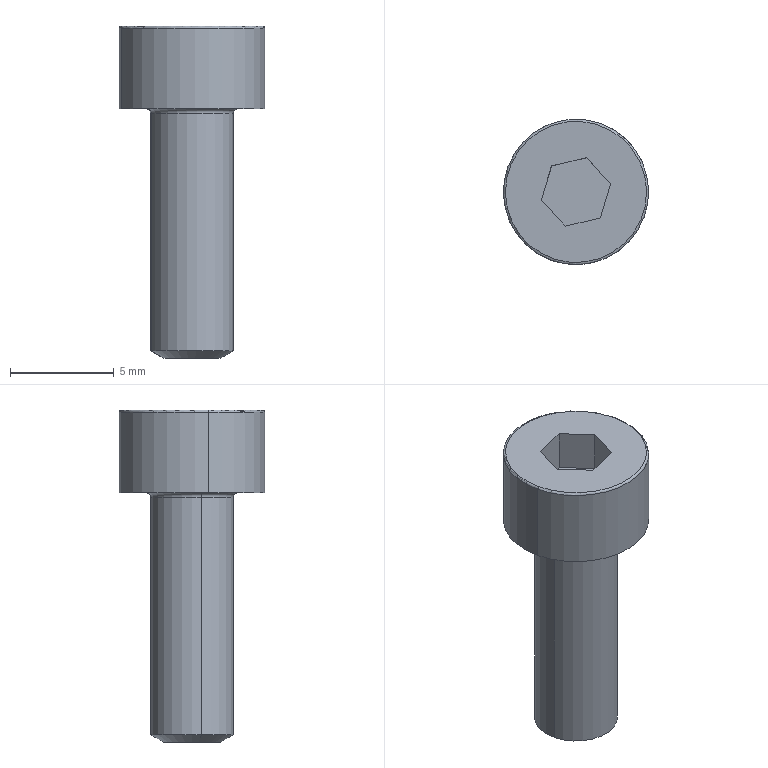Component | SolidWorks | MGL-PACK-01-00WeldedPlate1Assembly-1_SocketHeadCapScrew_M4_12[GB_T70.1-2000]-1 | 1 solid | 20 faces | box 7 x 7 x 16 mm | volume 288 mm3 | plane 10 | torus 4 | cylinder 4 | cone 2 | commonest cylinder face diameters 7 x2 4 x2
STEP:
#1=COLOUR_RGB('',0.7922,0.8196,0.9333);
#2=FILL_AREA_STYLE_COLOUR('',#1);
#3=FILL_AREA_STYLE('',(#2));
#4=SURFACE_STYLE_FILL_AREA(#3);
#5=SURFACE_SIDE_STYLE('',(#4));
#6=SURFACE_STYLE_USAGE(.BOTH.,#5);
#7=PRESENTATION_STYLE_ASSIGNMENT((#6));
#8=CARTESIAN_POINT('',(3.416,-2.272,0.3543));
#9=VERTEX_POINT('',#8);
#10=CARTESIAN_POINT('',(3.155,-2.334,0.3543));
#11=VERTEX_POINT('',#10);
#12=CARTESIAN_POINT('',(3.285,-2.303,0.3543));
#13=DIRECTION('',(0.,-0.,1.));
#14=DIRECTION('',(-0.9734,-0.2292,0.));
#15=AXIS2_PLACEMENT_3D('',#12,#13,#14);
#16=CIRCLE('',#15,0.1339);
#17=EDGE_CURVE('',#9,#11,#16,.T.);
#18=ORIENTED_EDGE('',*,*,#17,.F.);
#19=CARTESIAN_POINT('',(3.42,-2.272,0.3504));
#20=VERTEX_POINT('',#19);
#21=CARTESIAN_POINT('',(3.416,-2.272,0.3504));
#22=DIRECTION('',(-0.2292,0.9734,0.));
#23=DIRECTION('',(-0.9734,-0.2292,0.));
#24=AXIS2_PLACEMENT_3D('',#21,#22,#23);
#25=CIRCLE('',#24,0.003937);
#26=EDGE_CURVE('',#9,#20,#25,.T.);
#27=ORIENTED_EDGE('',*,*,#26,.T.);
#28=CARTESIAN_POINT('',(3.151,-2.335,0.3504));
#29=VERTEX_POINT('',#28);
#30=CARTESIAN_POINT('',(3.285,-2.303,0.3504));
#31=DIRECTION('',(0.,0.,-1.));
#32=DIRECTION('',(-0.9734,-0.2292,0.));
#33=AXIS2_PLACEMENT_3D('',#30,#31,#32);
#34=CIRCLE('',#33,0.1378);
#35=EDGE_CURVE('',#29,#20,#34,.T.);
#36=ORIENTED_EDGE('',*,*,#35,.F.);
#37=CARTESIAN_POINT('',(3.155,-2.334,0.3504));
#38=DIRECTION('',(0.2292,-0.9734,-0.));
#39=DIRECTION('',(0.9734,0.2292,0.));
#40=AXIS2_PLACEMENT_3D('',#37,#38,#39);
#41=CIRCLE('',#40,0.003937);
#42=EDGE_CURVE('',#11,#29,#41,.T.);
#43=ORIENTED_EDGE('',*,*,#42,.F.);
#44=EDGE_LOOP('',(#18,#27,#36,#43));
#45=FACE_OUTER_BOUND('',#44,.T.);
#46=CARTESIAN_POINT('',(3.285,-2.303,0.3504));
#47=DIRECTION('',(0.,0.,-1.));
#48=DIRECTION('',(-0.9734,-0.2292,-0.));
#49=AXIS2_PLACEMENT_3D('',#46,#47,#48);
#50=TOROIDAL_SURFACE('',#49,0.1339,0.003937);
#51=ADVANCED_FACE('',(#45),#50,.T.);
#52=CARTESIAN_POINT('',(3.339,-2.291,-0.2756));
#53=VERTEX_POINT('',#52);
#54=CARTESIAN_POINT('',(3.232,-2.316,-0.2756));
#55=VERTEX_POINT('',#54);
#56=CARTESIAN_POINT('',(3.285,-2.303,-0.2756));
#57=DIRECTION('',(0.,-0.,1.));
#58=DIRECTION('',(0.9734,0.2292,0.));
#59=AXIS2_PLACEMENT_3D('',#56,#57,#58);
#60=CIRCLE('',#59,0.05487);
#61=EDGE_CURVE('',#53,#55,#60,.T.);
#62=ORIENTED_EDGE('',*,*,#61,.T.);
#63=CARTESIAN_POINT('',(3.209,-2.321,-0.2618));
#64=VERTEX_POINT('',#63);
#65=CARTESIAN_POINT('',(3.209,-2.321,-0.2618));
#66=DIRECTION('',(-0.843,-0.1985,0.5));
#67=VECTOR('',#66,39.37);
#68=LINE('',#65,#67);
#69=EDGE_CURVE('',#55,#64,#68,.T.);
#70=ORIENTED_EDGE('',*,*,#69,.T.);
#71=CARTESIAN_POINT('',(3.362,-2.285,-0.2618));
#72=VERTEX_POINT('',#71);
#73=CARTESIAN_POINT('',(3.285,-2.303,-0.2618));
#74=DIRECTION('',(0.,-0.,1.));
#75=DIRECTION('',(0.9734,0.2292,0.));
#76=AXIS2_PLACEMENT_3D('',#73,#74,#75);
#77=CIRCLE('',#76,0.07874);
#78=EDGE_CURVE('',#72,#64,#77,.T.);
#79=ORIENTED_EDGE('',*,*,#78,.F.);
#80=CARTESIAN_POINT('',(3.362,-2.285,-0.2618));
#81=DIRECTION('',(0.843,0.1985,0.5));
#82=VECTOR('',#81,39.37);
#83=LINE('',#80,#82);
#84=EDGE_CURVE('',#53,#72,#83,.T.);
#85=ORIENTED_EDGE('',*,*,#84,.F.);
#86=EDGE_LOOP('',(#62,#70,#79,#85));
#87=FACE_OUTER_BOUND('',#86,.T.);
#88=CARTESIAN_POINT('',(3.285,-2.303,-0.2618));
#89=DIRECTION('',(0.,-0.,1.));
#90=DIRECTION('',(0.9734,0.2292,0.));
#91=AXIS2_PLACEMENT_3D('',#88,#89,#90);
#92=CONICAL_SURFACE('',#91,0.07874,1.047);
#93=ADVANCED_FACE('',(#87),#92,.T.);
#94=CARTESIAN_POINT('',(3.201,-2.323,0.1969));
#95=VERTEX_POINT('',#94);
#96=CARTESIAN_POINT('',(3.37,-2.283,0.1969));
#97=VERTEX_POINT('',#96);
#98=CARTESIAN_POINT('',(3.285,-2.303,0.1969));
#99=DIRECTION('',(0.,-0.,1.));
#100=DIRECTION('',(0.9734,0.2292,0.));
#101=AXIS2_PLACEMENT_3D('',#98,#99,#100);
#102=CIRCLE('',#101,0.08661);
#103=EDGE_CURVE('',#95,#97,#102,.T.);
#104=ORIENTED_EDGE('',*,*,#103,.F.);
#105=CARTESIAN_POINT('',(3.209,-2.321,0.189));
#106=VERTEX_POINT('',#105);
#107=CARTESIAN_POINT('',(3.201,-2.323,0.189));
#108=DIRECTION('',(-0.2292,0.9734,0.));
#109=DIRECTION('',(-0.9734,-0.2292,0.));
#110=AXIS2_PLACEMENT_3D('',#107,#108,#109);
#111=CIRCLE('',#110,0.007874);
#112=EDGE_CURVE('',#95,#106,#111,.T.);
#113=ORIENTED_EDGE('',*,*,#112,.T.);
#114=CARTESIAN_POINT('',(3.362,-2.285,0.189));
#115=VERTEX_POINT('',#114);
#116=CARTESIAN_POINT('',(3.285,-2.303,0.189));
#117=DIRECTION('',(0.,-0.,1.));
#118=DIRECTION('',(0.9734,0.2292,0.));
#119=AXIS2_PLACEMENT_3D('',#116,#117,#118);
#120=CIRCLE('',#119,0.07874);
#121=EDGE_CURVE('',#106,#115,#120,.T.);
#122=ORIENTED_EDGE('',*,*,#121,.T.);
#123=CARTESIAN_POINT('',(3.37,-2.283,0.189));
#124=DIRECTION('',(0.2292,-0.9734,-0.));
#125=DIRECTION('',(0.9734,0.2292,0.));
#126=AXIS2_PLACEMENT_3D('',#123,#124,#125);
#127=CIRCLE('',#126,0.007874);
#128=EDGE_CURVE('',#97,#115,#127,.T.);
#129=ORIENTED_EDGE('',*,*,#128,.F.);
#130=EDGE_LOOP('',(#104,#113,#122,#129));
#131=FACE_OUTER_BOUND('',#130,.T.);
#132=CARTESIAN_POINT('',(3.285,-2.303,0.189));
#133=DIRECTION('',(0.,-0.,1.));
#134=DIRECTION('',(0.9734,0.2292,0.));
#135=AXIS2_PLACEMENT_3D('',#132,#133,#134);
#136=TOROIDAL_SURFACE('',#135,0.08661,0.007874);
#137=ADVANCED_FACE('',(#131),#136,.F.);
#138=CARTESIAN_POINT('',(3.42,-2.272,0.1969));
#139=VERTEX_POINT('',#138);
#140=CARTESIAN_POINT('',(3.151,-2.335,0.1969));
#141=VERTEX_POINT('',#140);
#142=CARTESIAN_POINT('',(3.285,-2.303,0.1969));
#143=DIRECTION('',(0.,-0.,1.));
#144=DIRECTION('',(0.9734,0.2292,0.));
#145=AXIS2_PLACEMENT_3D('',#142,#143,#144);
#146=CIRCLE('',#145,0.1378);
#147=EDGE_CURVE('',#139,#141,#146,.T.);
#148=ORIENTED_EDGE('',*,*,#147,.T.);
#149=CARTESIAN_POINT('',(3.151,-2.335,0.3543));
#150=DIRECTION('',(0.,-0.,1.));
#151=VECTOR('',#150,39.37);
#152=LINE('',#149,#151);
#153=EDGE_CURVE('',#141,#29,#152,.T.);
#154=ORIENTED_EDGE('',*,*,#153,.T.);
#155=ORIENTED_EDGE('',*,*,#35,.T.);
#156=CARTESIAN_POINT('',(3.42,-2.272,0.3543));
#157=DIRECTION('',(0.,-0.,1.));
#158=VECTOR('',#157,39.37);
#159=LINE('',#156,#158);
#160=EDGE_CURVE('',#139,#20,#159,.T.);
#161=ORIENTED_EDGE('',*,*,#160,.F.);
#162=EDGE_LOOP('',(#148,#154,#155,#161));
#163=FACE_OUTER_BOUND('',#162,.T.);
#164=CARTESIAN_POINT('',(3.285,-2.303,0.3543));
#165=DIRECTION('',(0.,-0.,1.));
#166=DIRECTION('',(0.9734,0.2292,0.));
#167=AXIS2_PLACEMENT_3D('',#164,#165,#166);
#168=CYLINDRICAL_SURFACE('',#167,0.1378);
#169=ADVANCED_FACE('',(#163),#168,.T.);
#170=ORIENTED_EDGE('',*,*,#78,.T.);
#171=CARTESIAN_POINT('',(3.209,-2.321,0.3543));
#172=DIRECTION('',(0.,-0.,1.));
#173=VECTOR('',#172,39.37);
#174=LINE('',#171,#173);
#175=EDGE_CURVE('',#64,#106,#174,.T.);
#176=ORIENTED_EDGE('',*,*,#175,.T.);
#177=CARTESIAN_POINT('',(3.285,-2.303,0.189));
#178=DIRECTION('',(0.,-0.,1.));
#179=DIRECTION('',(0.9734,0.2292,0.));
#180=AXIS2_PLACEMENT_3D('',#177,#178,#179);
#181=CIRCLE('',#180,0.07874);
#182=EDGE_CURVE('',#115,#106,#181,.T.);
#183=ORIENTED_EDGE('',*,*,#182,.F.);
#184=CARTESIAN_POINT('',(3.362,-2.285,0.3543));
#185=DIRECTION('',(0.,-0.,1.));
#186=VECTOR('',#185,39.37);
#187=LINE('',#184,#186);
#188=EDGE_CURVE('',#72,#115,#187,.T.);
#189=ORIENTED_EDGE('',*,*,#188,.F.);
#190=EDGE_LOOP('',(#170,#176,#183,#189));
#191=FACE_OUTER_BOUND('',#190,.T.);
#192=CARTESIAN_POINT('',(3.285,-2.303,0.3543));
#193=DIRECTION('',(0.,-0.,1.));
#194=DIRECTION('',(0.9734,0.2292,0.));
#195=AXIS2_PLACEMENT_3D('',#192,#193,#194);
#196=CYLINDRICAL_SURFACE('',#195,0.07874);
#197=ADVANCED_FACE('',(#191),#196,.T.);
#198=ORIENTED_EDGE('',*,*,#175,.F.);
#199=CARTESIAN_POINT('',(3.285,-2.303,-0.2618));
#200=DIRECTION('',(0.,-0.,1.));
#201=DIRECTION('',(0.9734,0.2292,0.));
#202=AXIS2_PLACEMENT_3D('',#199,#200,#201);
#203=CIRCLE('',#202,0.07874);
#204=EDGE_CURVE('',#64,#72,#203,.T.);
#205=ORIENTED_EDGE('',*,*,#204,.T.);
#206=ORIENTED_EDGE('',*,*,#188,.T.);
#207=ORIENTED_EDGE('',*,*,#121,.F.);
#208=EDGE_LOOP('',(#198,#205,#206,#207));
#209=FACE_OUTER_BOUND('',#208,.T.);
#210=CARTESIAN_POINT('',(3.285,-2.303,0.3543));
#211=DIRECTION('',(0.,-0.,1.));
#212=DIRECTION('',(0.9734,0.2292,0.));
#213=AXIS2_PLACEMENT_3D('',#210,#211,#212);
#214=CYLINDRICAL_SURFACE('',#213,0.07874);
#215=ADVANCED_FACE('',(#209),#214,.T.);
#216=CARTESIAN_POINT('',(3.285,-2.303,0.3543));
#217=DIRECTION('',(0.,-0.,1.));
#218=DIRECTION('',(-0.9734,-0.2292,0.));
#219=AXIS2_PLACEMENT_3D('',#216,#217,#218);
#220=CIRCLE('',#219,0.1339);
#221=EDGE_CURVE('',#11,#9,#220,.T.);
#222=ORIENTED_EDGE('',*,*,#221,.T.);
#223=ORIENTED_EDGE('',*,*,#17,.T.);
#224=EDGE_LOOP('',(#222,#223));
#225=FACE_OUTER_BOUND('',#224,.T.);
#226=CARTESIAN_POINT('',(3.351,-2.288,0.3543));
#227=VERTEX_POINT('',#226);
#228=CARTESIAN_POINT('',(3.305,-2.238,0.3543));
#229=VERTEX_POINT('',#228);
#230=CARTESIAN_POINT('',(3.351,-2.288,0.3543));
#231=DIRECTION('',(-0.6852,0.7284,-0.));
#232=VECTOR('',#231,39.37);
#233=LINE('',#230,#232);
#234=EDGE_CURVE('',#227,#229,#233,.T.);
#235=ORIENTED_EDGE('',*,*,#234,.F.);
#236=CARTESIAN_POINT('',(3.332,-2.352,0.3543));
#237=VERTEX_POINT('',#236);
#238=CARTESIAN_POINT('',(3.332,-2.352,0.3543));
#239=DIRECTION('',(0.2882,0.9576,0.));
#240=VECTOR('',#239,39.37);
#241=LINE('',#238,#240);
#242=EDGE_CURVE('',#237,#227,#241,.T.);
#243=ORIENTED_EDGE('',*,*,#242,.F.);
#244=CARTESIAN_POINT('',(3.266,-2.368,0.3543));
#245=VERTEX_POINT('',#244);
#246=CARTESIAN_POINT('',(3.266,-2.368,0.3543));
#247=DIRECTION('',(0.9734,0.2292,0.));
#248=VECTOR('',#247,39.37);
#249=LINE('',#246,#248);
#250=EDGE_CURVE('',#245,#237,#249,.T.);
#251=ORIENTED_EDGE('',*,*,#250,.F.);
#252=CARTESIAN_POINT('',(3.22,-2.319,0.3543));
#253=VERTEX_POINT('',#252);
#254=CARTESIAN_POINT('',(3.22,-2.319,0.3543));
#255=DIRECTION('',(0.6852,-0.7284,0.));
#256=VECTOR('',#255,39.37);
#257=LINE('',#254,#256);
#258=EDGE_CURVE('',#253,#245,#257,.T.);
#259=ORIENTED_EDGE('',*,*,#258,.F.);
#260=CARTESIAN_POINT('',(3.239,-2.254,0.3543));
#261=VERTEX_POINT('',#260);
#262=CARTESIAN_POINT('',(3.239,-2.254,0.3543));
#263=DIRECTION('',(-0.2882,-0.9576,-0.));
#264=VECTOR('',#263,39.37);
#265=LINE('',#262,#264);
#266=EDGE_CURVE('',#261,#253,#265,.T.);
#267=ORIENTED_EDGE('',*,*,#266,.F.);
#268=CARTESIAN_POINT('',(3.305,-2.238,0.3543));
#269=DIRECTION('',(-0.9734,-0.2292,-0.));
#270=VECTOR('',#269,39.37);
#271=LINE('',#268,#270);
#272=EDGE_CURVE('',#229,#261,#271,.T.);
#273=ORIENTED_EDGE('',*,*,#272,.F.);
#274=EDGE_LOOP('',(#235,#243,#251,#259,#267,#273));
#275=FACE_BOUND('',#274,.T.);
#276=CARTESIAN_POINT('',(3.285,-2.303,0.3543));
#277=DIRECTION('',(0.,0.,-1.));
#278=DIRECTION('',(-0.9734,-0.2292,-0.));
#279=AXIS2_PLACEMENT_3D('',#276,#277,#278);
#280=PLANE('',#279);
#281=ADVANCED_FACE('',(#225,#275),#280,.F.);
#282=ORIENTED_EDGE('',*,*,#153,.F.);
#283=CARTESIAN_POINT('',(3.285,-2.303,0.1969));
#284=DIRECTION('',(0.,-0.,1.));
#285=DIRECTION('',(0.9734,0.2292,0.));
#286=AXIS2_PLACEMENT_3D('',#283,#284,#285);
#287=CIRCLE('',#286,0.1378);
#288=EDGE_CURVE('',#141,#139,#287,.T.);
#289=ORIENTED_EDGE('',*,*,#288,.T.);
#290=ORIENTED_EDGE('',*,*,#160,.T.);
#291=CARTESIAN_POINT('',(3.285,-2.303,0.3504));
#292=DIRECTION('',(0.,0.,-1.));
#293=DIRECTION('',(-0.9734,-0.2292,0.));
#294=AXIS2_PLACEMENT_3D('',#291,#292,#293);
#295=CIRCLE('',#294,0.1378);
#296=EDGE_CURVE('',#20,#29,#295,.T.);
#297=ORIENTED_EDGE('',*,*,#296,.T.);
#298=EDGE_LOOP('',(#282,#289,#290,#297));
#299=FACE_OUTER_BOUND('',#298,.T.);
#300=CARTESIAN_POINT('',(3.285,-2.303,0.3543));
#301=DIRECTION('',(0.,-0.,1.));
#302=DIRECTION('',(0.9734,0.2292,0.));
#303=AXIS2_PLACEMENT_3D('',#300,#301,#302);
#304=CYLINDRICAL_SURFACE('',#303,0.1378);
#305=ADVANCED_FACE('',(#299),#304,.T.);
#306=ORIENTED_EDGE('',*,*,#147,.F.);
#307=ORIENTED_EDGE('',*,*,#288,.F.);
#308=EDGE_LOOP('',(#306,#307));
#309=FACE_OUTER_BOUND('',#308,.T.);
#310=CARTESIAN_POINT('',(3.285,-2.303,0.1969));
#311=DIRECTION('',(0.,-0.,1.));
#312=DIRECTION('',(0.9734,0.2292,0.));
#313=AXIS2_PLACEMENT_3D('',#310,#311,#312);
#314=CIRCLE('',#313,0.08661);
#315=EDGE_CURVE('',#97,#95,#314,.T.);
#316=ORIENTED_EDGE('',*,*,#315,.T.);
#317=ORIENTED_EDGE('',*,*,#103,.T.);
#318=EDGE_LOOP('',(#316,#317));
#319=FACE_BOUND('',#318,.T.);
#320=CARTESIAN_POINT('',(3.254,-2.169,0.1969));
#321=DIRECTION('',(-0.,-0.,1.));
#322=DIRECTION('',(0.9734,0.2292,0.));
#323=AXIS2_PLACEMENT_3D('',#320,#321,#322);
#324=PLANE('',#323);
#325=ADVANCED_FACE('',(#309,#319),#324,.F.);
#326=ORIENTED_EDGE('',*,*,#112,.F.);
#327=ORIENTED_EDGE('',*,*,#315,.F.);
#328=ORIENTED_EDGE('',*,*,#128,.T.);
#329=ORIENTED_EDGE('',*,*,#182,.T.);
#330=EDGE_LOOP('',(#326,#327,#328,#329));
#331=FACE_OUTER_BOUND('',#330,.T.);
#332=CARTESIAN_POINT('',(3.285,-2.303,0.189));
#333=DIRECTION('',(0.,-0.,1.));
#334=DIRECTION('',(0.9734,0.2292,0.));
#335=AXIS2_PLACEMENT_3D('',#332,#333,#334);
#336=TOROIDAL_SURFACE('',#335,0.08661,0.007874);
#337=ADVANCED_FACE('',(#331),#336,.F.);
#338=ORIENTED_EDGE('',*,*,#242,.T.);
#339=CARTESIAN_POINT('',(3.351,-2.288,0.2756));
#340=VERTEX_POINT('',#339);
#341=CARTESIAN_POINT('',(3.351,-2.288,0.2756));
#342=DIRECTION('',(0.,-0.,1.));
#343=VECTOR('',#342,39.37);
#344=LINE('',#341,#343);
#345=EDGE_CURVE('',#340,#227,#344,.T.);
#346=ORIENTED_EDGE('',*,*,#345,.F.);
#347=CARTESIAN_POINT('',(3.332,-2.352,0.2756));
#348=VERTEX_POINT('',#347);
#349=CARTESIAN_POINT('',(3.332,-2.352,0.2756));
#350=DIRECTION('',(0.2882,0.9576,0.));
#351=VECTOR('',#350,39.37);
#352=LINE('',#349,#351);
#353=EDGE_CURVE('',#348,#340,#352,.T.);
#354=ORIENTED_EDGE('',*,*,#353,.F.);
#355=CARTESIAN_POINT('',(3.332,-2.352,0.2756));
#356=DIRECTION('',(0.,-0.,1.));
#357=VECTOR('',#356,39.37);
#358=LINE('',#355,#357);
#359=EDGE_CURVE('',#348,#237,#358,.T.);
#360=ORIENTED_EDGE('',*,*,#359,.T.);
#361=EDGE_LOOP('',(#338,#346,#354,#360));
#362=FACE_OUTER_BOUND('',#361,.T.);
#363=CARTESIAN_POINT('',(3.332,-2.352,0.2756));
#364=DIRECTION('',(0.9576,-0.2882,0.));
#365=DIRECTION('',(-0.2882,-0.9576,-0.));
#366=AXIS2_PLACEMENT_3D('',#363,#364,#365);
#367=PLANE('',#366);
#368=ADVANCED_FACE('',(#362),#367,.F.);
#369=ORIENTED_EDGE('',*,*,#250,.T.);
#370=ORIENTED_EDGE('',*,*,#359,.F.);
#371=CARTESIAN_POINT('',(3.266,-2.368,0.2756));
#372=VERTEX_POINT('',#371);
#373=CARTESIAN_POINT('',(3.266,-2.368,0.2756));
#374=DIRECTION('',(0.9734,0.2292,0.));
#375=VECTOR('',#374,39.37);
#376=LINE('',#373,#375);
#377=EDGE_CURVE('',#372,#348,#376,.T.);
#378=ORIENTED_EDGE('',*,*,#377,.F.);
#379=CARTESIAN_POINT('',(3.266,-2.368,0.2756));
#380=DIRECTION('',(0.,-0.,1.));
#381=VECTOR('',#380,39.37);
#382=LINE('',#379,#381);
#383=EDGE_CURVE('',#372,#245,#382,.T.);
#384=ORIENTED_EDGE('',*,*,#383,.T.);
#385=EDGE_LOOP('',(#369,#370,#378,#384));
#386=FACE_OUTER_BOUND('',#385,.T.);
#387=CARTESIAN_POINT('',(3.266,-2.368,0.2756));
#388=DIRECTION('',(0.2292,-0.9734,0.));
#389=DIRECTION('',(-0.9734,-0.2292,-0.));
#390=AXIS2_PLACEMENT_3D('',#387,#388,#389);
#391=PLANE('',#390);
#392=ADVANCED_FACE('',(#386),#391,.F.);
#393=ORIENTED_EDGE('',*,*,#258,.T.);
#394=ORIENTED_EDGE('',*,*,#383,.F.);
#395=CARTESIAN_POINT('',(3.22,-2.319,0.2756));
#396=VERTEX_POINT('',#395);
#397=CARTESIAN_POINT('',(3.22,-2.319,0.2756));
#398=DIRECTION('',(0.6852,-0.7284,0.));
#399=VECTOR('',#398,39.37);
#400=LINE('',#397,#399);
#401=EDGE_CURVE('',#396,#372,#400,.T.);
#402=ORIENTED_EDGE('',*,*,#401,.F.);
#403=CARTESIAN_POINT('',(3.22,-2.319,0.2756));
#404=DIRECTION('',(0.,-0.,1.));
#405=VECTOR('',#404,39.37);
#406=LINE('',#403,#405);
#407=EDGE_CURVE('',#396,#253,#406,.T.);
#408=ORIENTED_EDGE('',*,*,#407,.T.);
#409=EDGE_LOOP('',(#393,#394,#402,#408));
#410=FACE_OUTER_BOUND('',#409,.T.);
#411=CARTESIAN_POINT('',(3.22,-2.319,0.2756));
#412=DIRECTION('',(-0.7284,-0.6852,-0.));
#413=DIRECTION('',(-0.6852,0.7284,-0.));
#414=AXIS2_PLACEMENT_3D('',#411,#412,#413);
#415=PLANE('',#414);
#416=ADVANCED_FACE('',(#410),#415,.F.);
#417=ORIENTED_EDGE('',*,*,#266,.T.);
#418=ORIENTED_EDGE('',*,*,#407,.F.);
#419=CARTESIAN_POINT('',(3.239,-2.254,0.2756));
#420=VERTEX_POINT('',#419);
#421=CARTESIAN_POINT('',(3.239,-2.254,0.2756));
#422=DIRECTION('',(-0.2882,-0.9576,-0.));
#423=VECTOR('',#422,39.37);
#424=LINE('',#421,#423);
#425=EDGE_CURVE('',#420,#396,#424,.T.);
#426=ORIENTED_EDGE('',*,*,#425,.F.);
#427=CARTESIAN_POINT('',(3.239,-2.254,0.2756));
#428=DIRECTION('',(0.,-0.,1.));
#429=VECTOR('',#428,39.37);
#430=LINE('',#427,#429);
#431=EDGE_CURVE('',#420,#261,#430,.T.);
#432=ORIENTED_EDGE('',*,*,#431,.T.);
#433=EDGE_LOOP('',(#417,#418,#426,#432));
#434=FACE_OUTER_BOUND('',#433,.T.);
#435=CARTESIAN_POINT('',(3.239,-2.254,0.2756));
#436=DIRECTION('',(-0.9576,0.2882,-0.));
#437=DIRECTION('',(0.2882,0.9576,0.));
#438=AXIS2_PLACEMENT_3D('',#435,#436,#437);
#439=PLANE('',#438);
#440=ADVANCED_FACE('',(#434),#439,.F.);
#441=ORIENTED_EDGE('',*,*,#272,.T.);
#442=ORIENTED_EDGE('',*,*,#431,.F.);
#443=CARTESIAN_POINT('',(3.305,-2.238,0.2756));
#444=VERTEX_POINT('',#443);
#445=CARTESIAN_POINT('',(3.305,-2.238,0.2756));
#446=DIRECTION('',(-0.9734,-0.2292,-0.));
#447=VECTOR('',#446,39.37);
#448=LINE('',#445,#447);
#449=EDGE_CURVE('',#444,#420,#448,.T.);
#450=ORIENTED_EDGE('',*,*,#449,.F.);
#451=CARTESIAN_POINT('',(3.305,-2.238,0.2756));
#452=DIRECTION('',(0.,-0.,1.));
#453=VECTOR('',#452,39.37);
#454=LINE('',#451,#453);
#455=EDGE_CURVE('',#444,#229,#454,.T.);
#456=ORIENTED_EDGE('',*,*,#455,.T.);
#457=EDGE_LOOP('',(#441,#442,#450,#456));
#458=FACE_OUTER_BOUND('',#457,.T.);
#459=CARTESIAN_POINT('',(3.305,-2.238,0.2756));
#460=DIRECTION('',(-0.2292,0.9734,0.));
#461=DIRECTION('',(0.9734,0.2292,0.));
#462=AXIS2_PLACEMENT_3D('',#459,#460,#461);
#463=PLANE('',#462);
#464=ADVANCED_FACE('',(#458),#463,.F.);
#465=ORIENTED_EDGE('',*,*,#234,.T.);
#466=ORIENTED_EDGE('',*,*,#455,.F.);
#467=CARTESIAN_POINT('',(3.351,-2.288,0.2756));
#468=DIRECTION('',(-0.6852,0.7284,-0.));
#469=VECTOR('',#468,39.37);
#470=LINE('',#467,#469);
#471=EDGE_CURVE('',#340,#444,#470,.T.);
#472=ORIENTED_EDGE('',*,*,#471,.F.);
#473=ORIENTED_EDGE('',*,*,#345,.T.);
#474=EDGE_LOOP('',(#465,#466,#472,#473));
#475=FACE_OUTER_BOUND('',#474,.T.);
#476=CARTESIAN_POINT('',(3.351,-2.288,0.2756));
#477=DIRECTION('',(0.7284,0.6852,0.));
#478=DIRECTION('',(0.6852,-0.7284,0.));
#479=AXIS2_PLACEMENT_3D('',#476,#477,#478);
#480=PLANE('',#479);
#481=ADVANCED_FACE('',(#475),#480,.F.);
#482=ORIENTED_EDGE('',*,*,#353,.T.);
#483=ORIENTED_EDGE('',*,*,#471,.T.);
#484=ORIENTED_EDGE('',*,*,#449,.T.);
#485=ORIENTED_EDGE('',*,*,#425,.T.);
#486=ORIENTED_EDGE('',*,*,#401,.T.);
#487=ORIENTED_EDGE('',*,*,#377,.T.);
#488=EDGE_LOOP('',(#482,#483,#484,#485,#486,#487));
#489=FACE_OUTER_BOUND('',#488,.T.);
#490=CARTESIAN_POINT('',(3.371,-2.223,0.2756));
#491=DIRECTION('',(-0.,-0.,1.));
#492=DIRECTION('',(0.9734,0.2292,0.));
#493=AXIS2_PLACEMENT_3D('',#490,#491,#492);
#494=PLANE('',#493);
#495=ADVANCED_FACE('',(#489),#494,.T.);
#496=ORIENTED_EDGE('',*,*,#69,.F.);
#497=CARTESIAN_POINT('',(3.285,-2.303,-0.2756));
#498=DIRECTION('',(0.,-0.,1.));
#499=DIRECTION('',(0.9734,0.2292,0.));
#500=AXIS2_PLACEMENT_3D('',#497,#498,#499);
#501=CIRCLE('',#500,0.05487);
#502=EDGE_CURVE('',#55,#53,#501,.T.);
#503=ORIENTED_EDGE('',*,*,#502,.T.);
#504=ORIENTED_EDGE('',*,*,#84,.T.);
#505=ORIENTED_EDGE('',*,*,#204,.F.);
#506=EDGE_LOOP('',(#496,#503,#504,#505));
#507=FACE_OUTER_BOUND('',#506,.T.);
#508=CARTESIAN_POINT('',(3.285,-2.303,-0.2618));
#509=DIRECTION('',(0.,-0.,1.));
#510=DIRECTION('',(0.9734,0.2292,0.));
#511=AXIS2_PLACEMENT_3D('',#508,#509,#510);
#512=CONICAL_SURFACE('',#511,0.07874,1.047);
#513=ADVANCED_FACE('',(#507),#512,.T.);
#514=ORIENTED_EDGE('',*,*,#61,.F.);
#515=ORIENTED_EDGE('',*,*,#502,.F.);
#516=EDGE_LOOP('',(#514,#515));
#517=FACE_OUTER_BOUND('',#516,.T.);
#518=CARTESIAN_POINT('',(3.267,-2.227,-0.2756));
#519=DIRECTION('',(-0.,-0.,1.));
#520=DIRECTION('',(0.9734,0.2292,0.));
#521=AXIS2_PLACEMENT_3D('',#518,#519,#520);
#522=PLANE('',#521);
#523=ADVANCED_FACE('',(#517),#522,.F.);
#524=ORIENTED_EDGE('',*,*,#26,.F.);
#525=ORIENTED_EDGE('',*,*,#221,.F.);
#526=ORIENTED_EDGE('',*,*,#42,.T.);
#527=ORIENTED_EDGE('',*,*,#296,.F.);
#528=EDGE_LOOP('',(#524,#525,#526,#527));
#529=FACE_OUTER_BOUND('',#528,.T.);
#530=CARTESIAN_POINT('',(3.285,-2.303,0.3504));
#531=DIRECTION('',(0.,0.,-1.));
#532=DIRECTION('',(-0.9734,-0.2292,-0.));
#533=AXIS2_PLACEMENT_3D('',#530,#531,#532);
#534=TOROIDAL_SURFACE('',#533,0.1339,0.003937);
#535=ADVANCED_FACE('',(#529),#534,.T.);
#536=CLOSED_SHELL('',(#51,#93,#137,#169,#197,#215,#281,#305,#325,#337,#368,#392,#416,#440,#464,#481,#495,#513,#523,#535));
#537=MANIFOLD_SOLID_BREP('',#536);
#538=STYLED_ITEM('',(#7),#537);
#539=PRESENTATION_LAYER_ASSIGNMENT('','',(#538));
#540=CARTESIAN_POINT('',(0.,0.,0.));
#541=DIRECTION('',(0.,0.,1.));
#542=DIRECTION('',(1.,0.,0.));
#543=AXIS2_PLACEMENT_3D('',#540,#541,#542);
#544=(LENGTH_UNIT()NAMED_UNIT(*)SI_UNIT($,.METRE.));
#545=LENGTH_MEASURE_WITH_UNIT(LENGTH_MEASURE(0.0254),#544);
#546=DIMENSIONAL_EXPONENTS(1.,0.,0.,0.,0.,0.,0.);
#547=(CONVERSION_BASED_UNIT('',#545)LENGTH_UNIT()NAMED_UNIT(#546));
#548=UNCERTAINTY_MEASURE_WITH_UNIT(LENGTH_MEASURE(0.00001),#547,'','');
#549=(NAMED_UNIT(*)PLANE_ANGLE_UNIT()SI_UNIT($,.RADIAN.));
#550=(NAMED_UNIT(*)SI_UNIT($,.STERADIAN.)SOLID_ANGLE_UNIT());
#551=(GEOMETRIC_REPRESENTATION_CONTEXT(3)GLOBAL_UNCERTAINTY_ASSIGNED_CONTEXT((#548))GLOBAL_UNIT_ASSIGNED_CONTEXT((#547,#549,#550))REPRESENTATION_CONTEXT('',''));
#552=ADVANCED_BREP_SHAPE_REPRESENTATION('',(#537,#543),#551);
#553=(LENGTH_UNIT()NAMED_UNIT(*)SI_UNIT($,.METRE.));
#554=LENGTH_MEASURE_WITH_UNIT(LENGTH_MEASURE(0.0254),#553);
#555=DIMENSIONAL_EXPONENTS(1.,0.,0.,0.,0.,0.,0.);
#556=(CONVERSION_BASED_UNIT('',#554)LENGTH_UNIT()NAMED_UNIT(#555));
#557=UNCERTAINTY_MEASURE_WITH_UNIT(LENGTH_MEASURE(0.00001),#556,'','');
#558=(NAMED_UNIT(*)PLANE_ANGLE_UNIT()SI_UNIT($,.RADIAN.));
#559=(NAMED_UNIT(*)SI_UNIT($,.STERADIAN.)SOLID_ANGLE_UNIT());
#560=(GEOMETRIC_REPRESENTATION_CONTEXT(3)GLOBAL_UNCERTAINTY_ASSIGNED_CONTEXT((#557))GLOBAL_UNIT_ASSIGNED_CONTEXT((#556,#558,#559))REPRESENTATION_CONTEXT('',''));
#561=MECHANICAL_DESIGN_GEOMETRIC_PRESENTATION_REPRESENTATION('',(#538),#560);